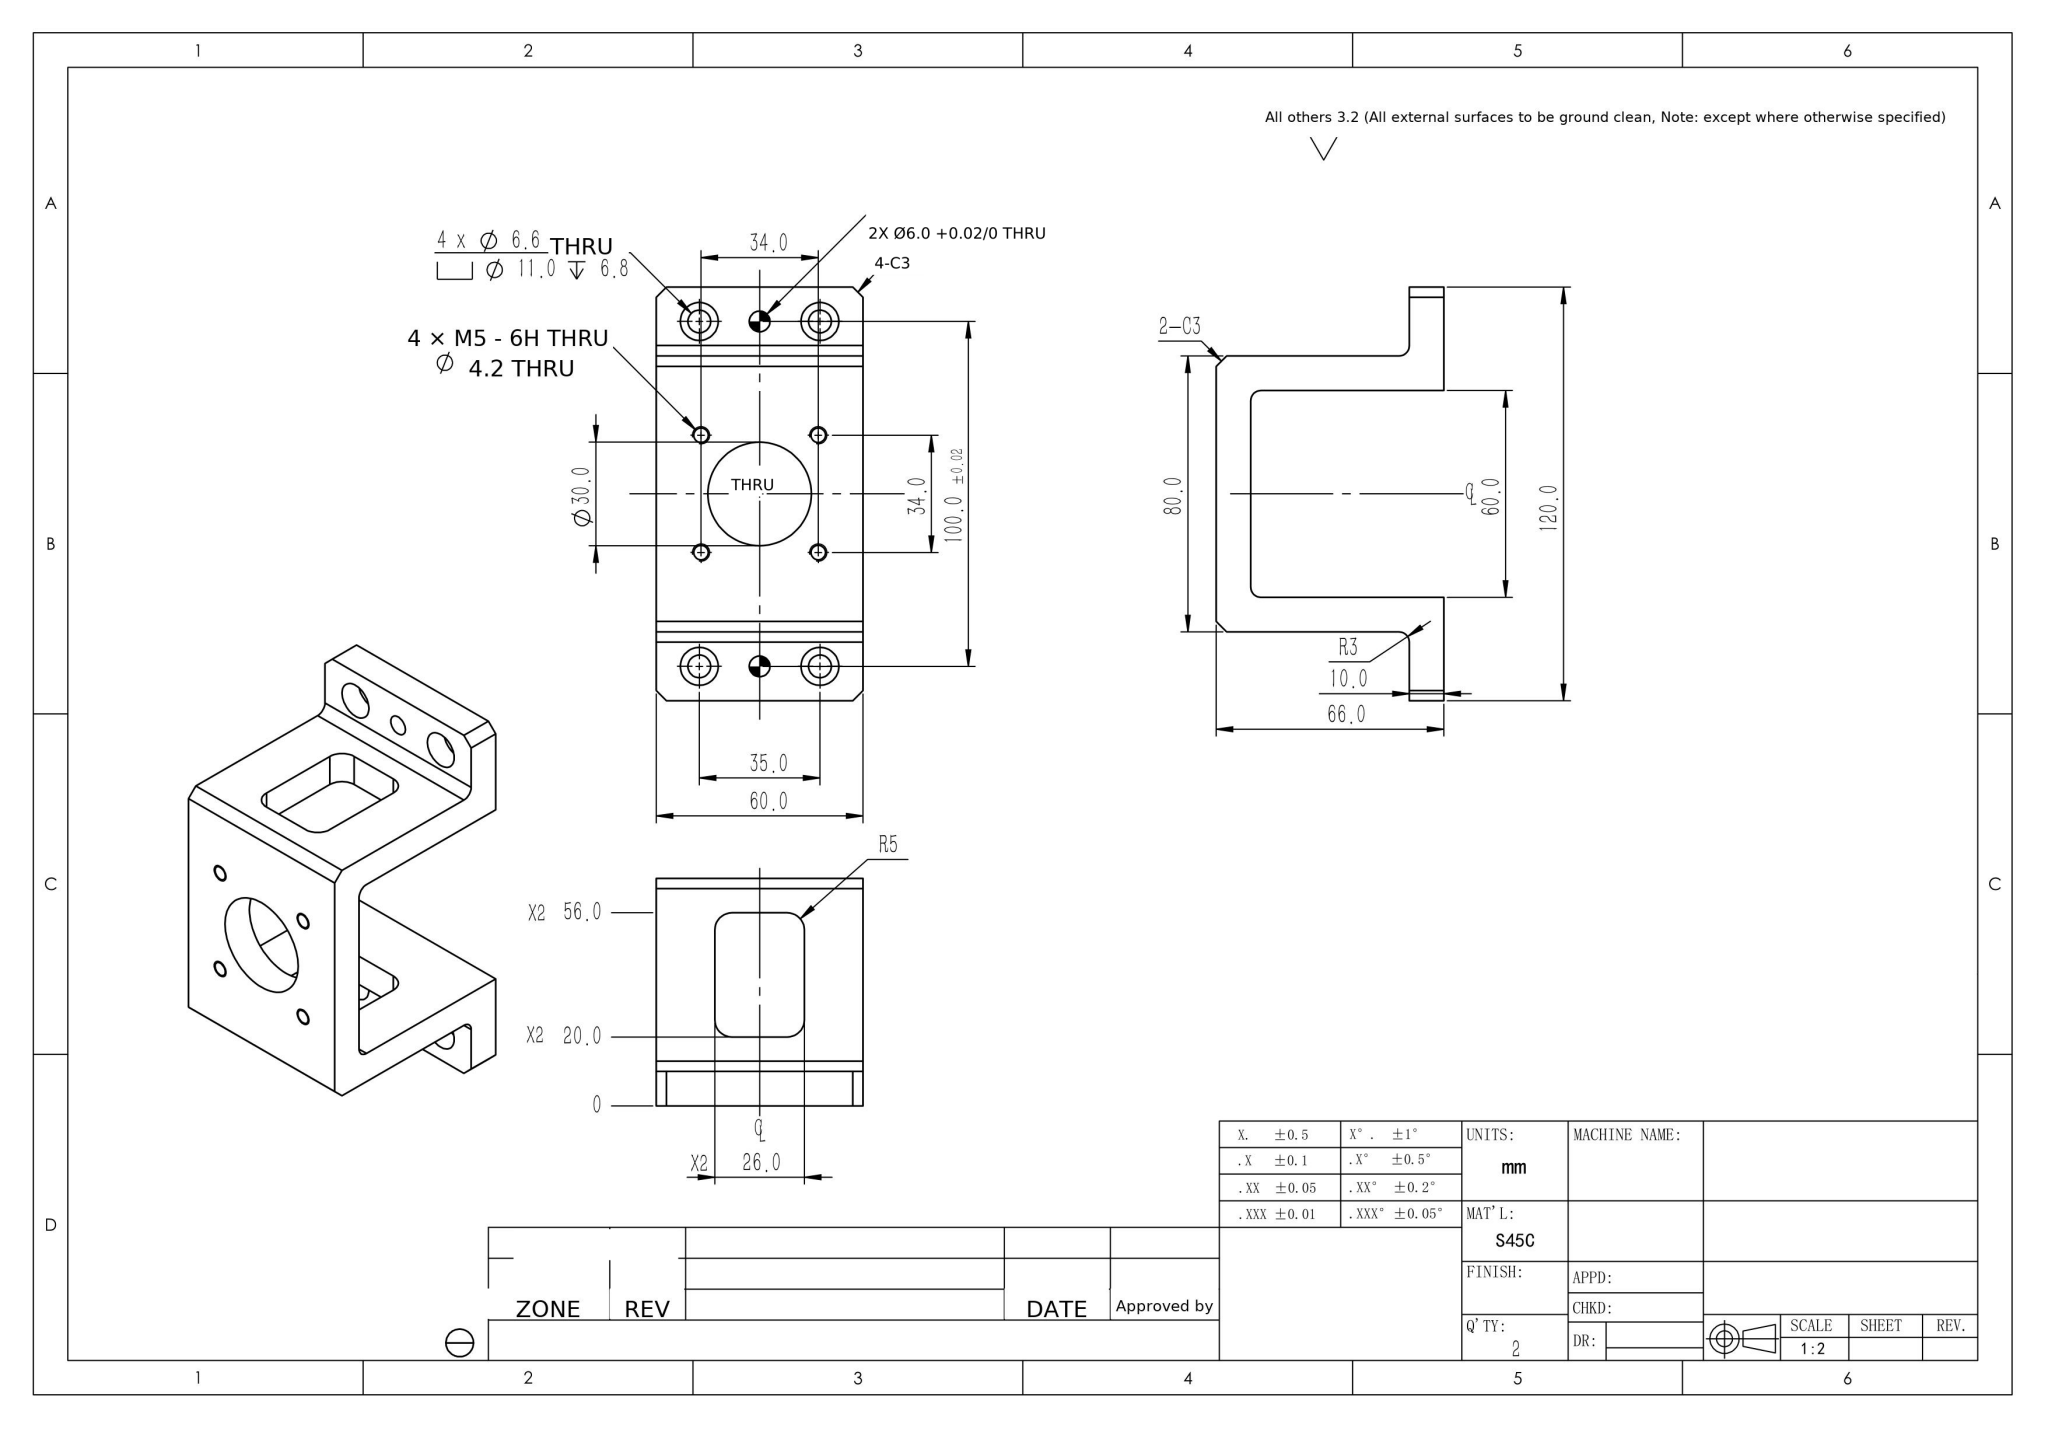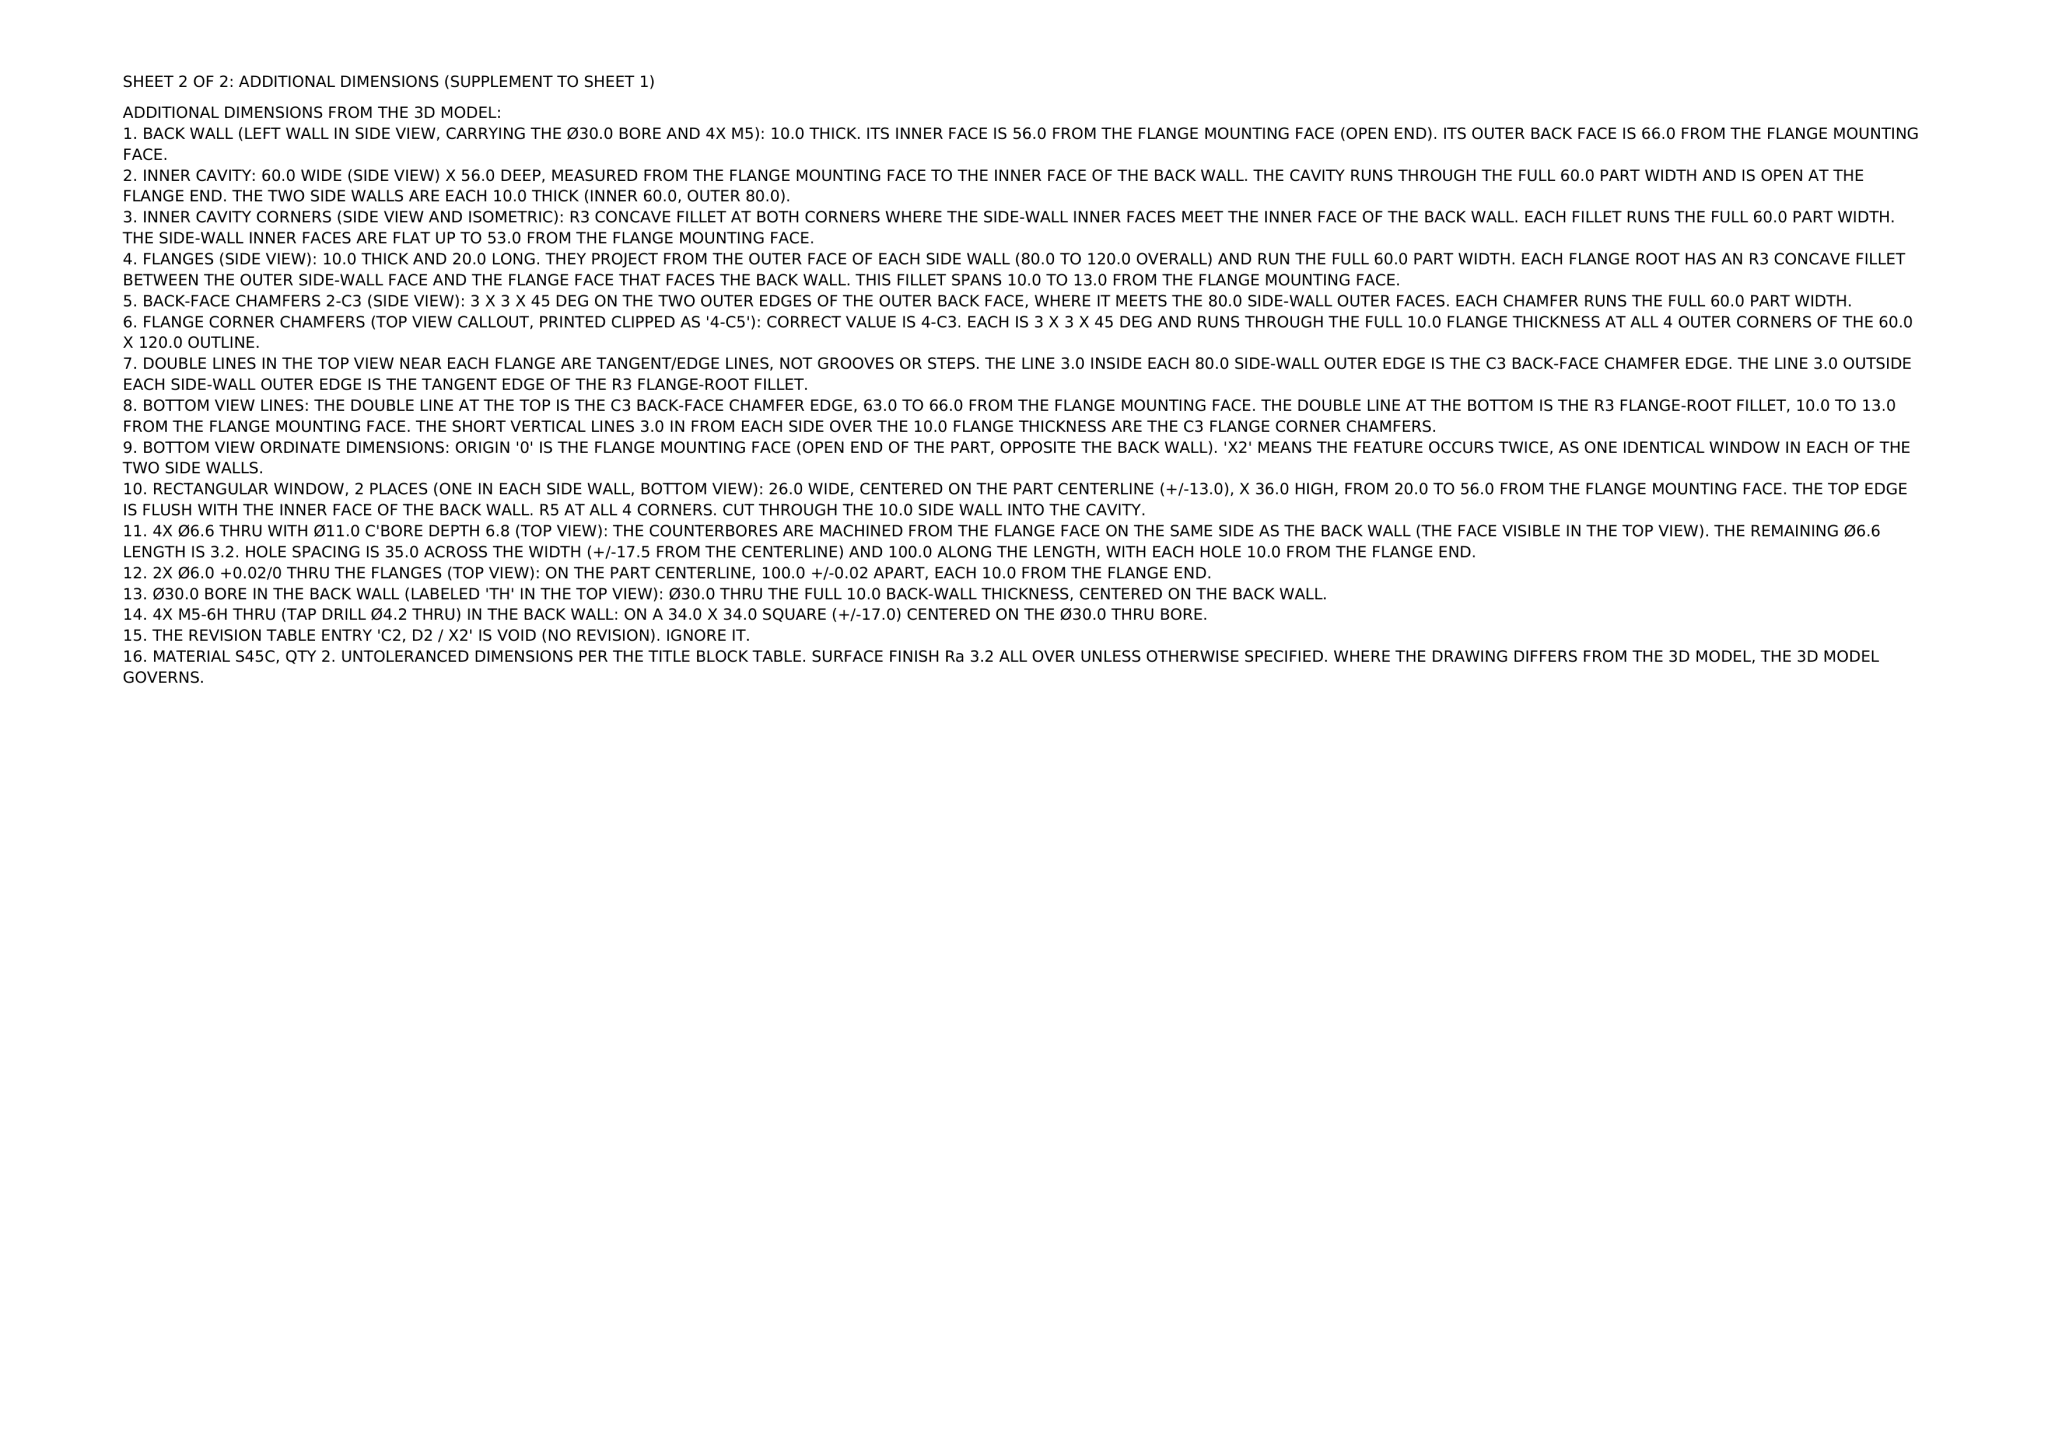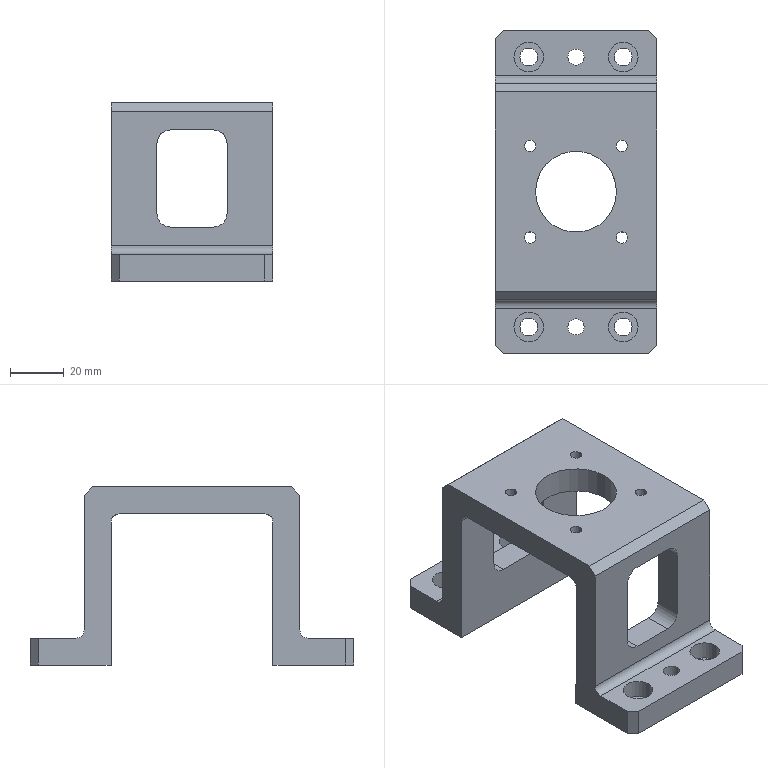Part | NX | mm | Elevated Motor Mounting Bracket | 1 solid | 74 faces | box 60 x 120 x 66 mm | volume 109363 mm3 | cylinder 44 | plane 30 | commonest cylinder face diameters 6 x10 11 x8 6.6 x8 4.2 x8 10 x8 30 x2